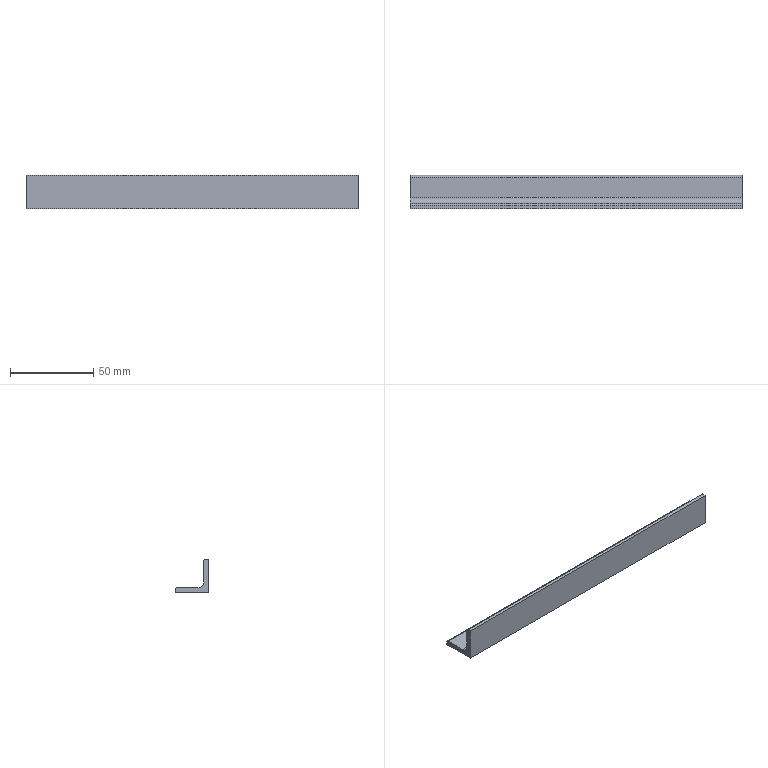Component | SolidWorks | hot-rolled equal angle gb-6 | 1 solid | 11 faces | box 200 x 20 x 20 mm | volume 22640 mm3 | plane 8 | cylinder 3 | commonest cylinder face diameters 2 x2 7 x1
build123d program:
from build123d import *

# Parameters (mm, degrees)
BASE_DEPTH = 200


with BuildPart() as part:
    # Sketch1 → Base (new body)
    with BuildSketch(Plane.YZ):
        with BuildLine():
            Line((0, 20), (0, 0))
            Line((0, 0), (20, 0))
            Line((20, 0), (20, 2))
            ThreePointArc((20, 2), (19.707, 2.707), (19, 3))
            Line((19, 3), (6.5, 3))
            ThreePointArc((6.5, 3), (4.025, 4.025), (3, 6.5))
            Line((3, 6.5), (3, 19))
            ThreePointArc((3, 19), (2.707, 19.707), (2, 20))
            Line((2, 20), (0, 20))
        make_face()
    extrude(amount=BASE_DEPTH)


solid = part.part

# Placed as in the assembly
solid = solid.moved(Location((-40, 537, -215), (0, 0, 0)))
STEP:
#1=CARTESIAN_POINT('',(-1.575,21.22,-7.677));
#2=VERTEX_POINT('',#1);
#3=CARTESIAN_POINT('',(-1.575,21.142,-7.677));
#4=VERTEX_POINT('',#3);
#5=CARTESIAN_POINT('',(-1.575,21.142,-7.677));
#6=DIRECTION('',(0.,-1.,-0.));
#7=VECTOR('',#6,39.37);
#8=LINE('',#5,#7);
#9=EDGE_CURVE('',#2,#4,#8,.T.);
#10=ORIENTED_EDGE('',*,*,#9,.T.);
#11=CARTESIAN_POINT('',(6.299,21.142,-7.677));
#12=VERTEX_POINT('',#11);
#13=CARTESIAN_POINT('',(6.299,21.142,-7.677));
#14=DIRECTION('',(-1.,0.,0.));
#15=VECTOR('',#14,39.37);
#16=LINE('',#13,#15);
#17=EDGE_CURVE('',#12,#4,#16,.T.);
#18=ORIENTED_EDGE('',*,*,#17,.F.);
#19=CARTESIAN_POINT('',(6.299,21.22,-7.677));
#20=VERTEX_POINT('',#19);
#21=CARTESIAN_POINT('',(6.299,21.142,-7.677));
#22=DIRECTION('',(0.,-1.,-0.));
#23=VECTOR('',#22,39.37);
#24=LINE('',#21,#23);
#25=EDGE_CURVE('',#20,#12,#24,.T.);
#26=ORIENTED_EDGE('',*,*,#25,.F.);
#27=CARTESIAN_POINT('',(6.299,21.22,-7.677));
#28=DIRECTION('',(-1.,0.,0.));
#29=VECTOR('',#28,39.37);
#30=LINE('',#27,#29);
#31=EDGE_CURVE('',#20,#2,#30,.T.);
#32=ORIENTED_EDGE('',*,*,#31,.T.);
#33=EDGE_LOOP('',(#10,#18,#26,#32));
#34=FACE_OUTER_BOUND('',#33,.T.);
#35=CARTESIAN_POINT('',(6.299,21.142,-7.677));
#36=DIRECTION('',(0.,0.,-1.));
#37=DIRECTION('',(0.,1.,0.));
#38=AXIS2_PLACEMENT_3D('',#35,#36,#37);
#39=PLANE('',#38);
#40=ADVANCED_FACE('',(#34),#39,.F.);
#41=CARTESIAN_POINT('',(-1.575,21.142,-8.465));
#42=VERTEX_POINT('',#41);
#43=CARTESIAN_POINT('',(-1.575,21.142,-7.677));
#44=DIRECTION('',(0.,-0.,-1.));
#45=VECTOR('',#44,39.37);
#46=LINE('',#43,#45);
#47=EDGE_CURVE('',#4,#42,#46,.T.);
#48=ORIENTED_EDGE('',*,*,#47,.T.);
#49=CARTESIAN_POINT('',(6.299,21.142,-8.465));
#50=VERTEX_POINT('',#49);
#51=CARTESIAN_POINT('',(6.299,21.142,-8.465));
#52=DIRECTION('',(-1.,0.,0.));
#53=VECTOR('',#52,39.37);
#54=LINE('',#51,#53);
#55=EDGE_CURVE('',#50,#42,#54,.T.);
#56=ORIENTED_EDGE('',*,*,#55,.F.);
#57=CARTESIAN_POINT('',(6.299,21.142,-7.677));
#58=DIRECTION('',(0.,-0.,-1.));
#59=VECTOR('',#58,39.37);
#60=LINE('',#57,#59);
#61=EDGE_CURVE('',#12,#50,#60,.T.);
#62=ORIENTED_EDGE('',*,*,#61,.F.);
#63=ORIENTED_EDGE('',*,*,#17,.T.);
#64=EDGE_LOOP('',(#48,#56,#62,#63));
#65=FACE_OUTER_BOUND('',#64,.T.);
#66=CARTESIAN_POINT('',(6.299,21.142,-7.677));
#67=DIRECTION('',(0.,1.,-0.));
#68=DIRECTION('',(0.,0.,1.));
#69=AXIS2_PLACEMENT_3D('',#66,#67,#68);
#70=PLANE('',#69);
#71=ADVANCED_FACE('',(#65),#70,.F.);
#72=CARTESIAN_POINT('',(-1.575,21.929,-8.465));
#73=VERTEX_POINT('',#72);
#74=CARTESIAN_POINT('',(-1.575,21.142,-8.465));
#75=DIRECTION('',(0.,1.,0.));
#76=VECTOR('',#75,39.37);
#77=LINE('',#74,#76);
#78=EDGE_CURVE('',#42,#73,#77,.T.);
#79=ORIENTED_EDGE('',*,*,#78,.T.);
#80=CARTESIAN_POINT('',(6.299,21.929,-8.465));
#81=VERTEX_POINT('',#80);
#82=CARTESIAN_POINT('',(6.299,21.929,-8.465));
#83=DIRECTION('',(-1.,0.,0.));
#84=VECTOR('',#83,39.37);
#85=LINE('',#82,#84);
#86=EDGE_CURVE('',#81,#73,#85,.T.);
#87=ORIENTED_EDGE('',*,*,#86,.F.);
#88=CARTESIAN_POINT('',(6.299,21.142,-8.465));
#89=DIRECTION('',(0.,1.,0.));
#90=VECTOR('',#89,39.37);
#91=LINE('',#88,#90);
#92=EDGE_CURVE('',#50,#81,#91,.T.);
#93=ORIENTED_EDGE('',*,*,#92,.F.);
#94=ORIENTED_EDGE('',*,*,#55,.T.);
#95=EDGE_LOOP('',(#79,#87,#93,#94));
#96=FACE_OUTER_BOUND('',#95,.T.);
#97=CARTESIAN_POINT('',(6.299,21.142,-8.465));
#98=DIRECTION('',(0.,0.,1.));
#99=DIRECTION('',(1.,0.,0.));
#100=AXIS2_PLACEMENT_3D('',#97,#98,#99);
#101=PLANE('',#100);
#102=ADVANCED_FACE('',(#96),#101,.F.);
#103=CARTESIAN_POINT('',(-1.575,21.929,-8.386));
#104=VERTEX_POINT('',#103);
#105=CARTESIAN_POINT('',(-1.575,21.929,-8.465));
#106=DIRECTION('',(0.,0.,1.));
#107=VECTOR('',#106,39.37);
#108=LINE('',#105,#107);
#109=EDGE_CURVE('',#73,#104,#108,.T.);
#110=ORIENTED_EDGE('',*,*,#109,.T.);
#111=CARTESIAN_POINT('',(6.299,21.929,-8.386));
#112=VERTEX_POINT('',#111);
#113=CARTESIAN_POINT('',(6.299,21.929,-8.386));
#114=DIRECTION('',(-1.,0.,0.));
#115=VECTOR('',#114,39.37);
#116=LINE('',#113,#115);
#117=EDGE_CURVE('',#112,#104,#116,.T.);
#118=ORIENTED_EDGE('',*,*,#117,.F.);
#119=CARTESIAN_POINT('',(6.299,21.929,-8.465));
#120=DIRECTION('',(0.,0.,1.));
#121=VECTOR('',#120,39.37);
#122=LINE('',#119,#121);
#123=EDGE_CURVE('',#81,#112,#122,.T.);
#124=ORIENTED_EDGE('',*,*,#123,.F.);
#125=ORIENTED_EDGE('',*,*,#86,.T.);
#126=EDGE_LOOP('',(#110,#118,#124,#125));
#127=FACE_OUTER_BOUND('',#126,.T.);
#128=CARTESIAN_POINT('',(6.299,21.929,-8.465));
#129=DIRECTION('',(0.,-1.,0.));
#130=DIRECTION('',(0.,-0.,-1.));
#131=AXIS2_PLACEMENT_3D('',#128,#129,#130);
#132=PLANE('',#131);
#133=ADVANCED_FACE('',(#127),#132,.F.);
#134=CARTESIAN_POINT('',(-1.575,21.89,-8.346));
#135=VERTEX_POINT('',#134);
#136=CARTESIAN_POINT('',(-1.575,21.89,-8.386));
#137=DIRECTION('',(1.,0.,0.));
#138=DIRECTION('',(0.,0.,-1.));
#139=AXIS2_PLACEMENT_3D('',#136,#137,#138);
#140=CIRCLE('',#139,0.03937);
#141=EDGE_CURVE('',#104,#135,#140,.T.);
#142=ORIENTED_EDGE('',*,*,#141,.T.);
#143=CARTESIAN_POINT('',(6.299,21.89,-8.346));
#144=VERTEX_POINT('',#143);
#145=CARTESIAN_POINT('',(6.299,21.89,-8.346));
#146=DIRECTION('',(-1.,0.,0.));
#147=VECTOR('',#146,39.37);
#148=LINE('',#145,#147);
#149=EDGE_CURVE('',#144,#135,#148,.T.);
#150=ORIENTED_EDGE('',*,*,#149,.F.);
#151=CARTESIAN_POINT('',(6.299,21.89,-8.386));
#152=DIRECTION('',(1.,0.,0.));
#153=DIRECTION('',(0.,0.,-1.));
#154=AXIS2_PLACEMENT_3D('',#151,#152,#153);
#155=CIRCLE('',#154,0.03937);
#156=EDGE_CURVE('',#112,#144,#155,.T.);
#157=ORIENTED_EDGE('',*,*,#156,.F.);
#158=ORIENTED_EDGE('',*,*,#117,.T.);
#159=EDGE_LOOP('',(#142,#150,#157,#158));
#160=FACE_OUTER_BOUND('',#159,.T.);
#161=CARTESIAN_POINT('',(6.299,21.89,-8.386));
#162=DIRECTION('',(-1.,0.,0.));
#163=DIRECTION('',(0.,0.,1.));
#164=AXIS2_PLACEMENT_3D('',#161,#162,#163);
#165=CYLINDRICAL_SURFACE('',#164,0.03937);
#166=ADVANCED_FACE('',(#160),#165,.T.);
#167=CARTESIAN_POINT('',(-1.575,21.398,-8.346));
#168=VERTEX_POINT('',#167);
#169=CARTESIAN_POINT('',(-1.575,21.398,-8.346));
#170=DIRECTION('',(0.,-1.,0.));
#171=VECTOR('',#170,39.37);
#172=LINE('',#169,#171);
#173=EDGE_CURVE('',#135,#168,#172,.T.);
#174=ORIENTED_EDGE('',*,*,#173,.T.);
#175=CARTESIAN_POINT('',(6.299,21.398,-8.346));
#176=VERTEX_POINT('',#175);
#177=CARTESIAN_POINT('',(6.299,21.398,-8.346));
#178=DIRECTION('',(-1.,0.,0.));
#179=VECTOR('',#178,39.37);
#180=LINE('',#177,#179);
#181=EDGE_CURVE('',#176,#168,#180,.T.);
#182=ORIENTED_EDGE('',*,*,#181,.F.);
#183=CARTESIAN_POINT('',(6.299,21.398,-8.346));
#184=DIRECTION('',(0.,-1.,0.));
#185=VECTOR('',#184,39.37);
#186=LINE('',#183,#185);
#187=EDGE_CURVE('',#144,#176,#186,.T.);
#188=ORIENTED_EDGE('',*,*,#187,.F.);
#189=ORIENTED_EDGE('',*,*,#149,.T.);
#190=EDGE_LOOP('',(#174,#182,#188,#189));
#191=FACE_OUTER_BOUND('',#190,.T.);
#192=CARTESIAN_POINT('',(6.299,21.398,-8.346));
#193=DIRECTION('',(0.,-0.,-1.));
#194=DIRECTION('',(0.,1.,-0.));
#195=AXIS2_PLACEMENT_3D('',#192,#193,#194);
#196=PLANE('',#195);
#197=ADVANCED_FACE('',(#191),#196,.F.);
#198=CARTESIAN_POINT('',(-1.575,21.26,-8.209));
#199=VERTEX_POINT('',#198);
#200=CARTESIAN_POINT('',(-1.575,21.398,-8.209));
#201=DIRECTION('',(-1.,0.,0.));
#202=DIRECTION('',(0.,0.,-1.));
#203=AXIS2_PLACEMENT_3D('',#200,#201,#202);
#204=CIRCLE('',#203,0.1378);
#205=EDGE_CURVE('',#168,#199,#204,.T.);
#206=ORIENTED_EDGE('',*,*,#205,.T.);
#207=CARTESIAN_POINT('',(6.299,21.26,-8.209));
#208=VERTEX_POINT('',#207);
#209=CARTESIAN_POINT('',(6.299,21.26,-8.209));
#210=DIRECTION('',(-1.,0.,0.));
#211=VECTOR('',#210,39.37);
#212=LINE('',#209,#211);
#213=EDGE_CURVE('',#208,#199,#212,.T.);
#214=ORIENTED_EDGE('',*,*,#213,.F.);
#215=CARTESIAN_POINT('',(6.299,21.398,-8.209));
#216=DIRECTION('',(-1.,0.,0.));
#217=DIRECTION('',(0.,0.,-1.));
#218=AXIS2_PLACEMENT_3D('',#215,#216,#217);
#219=CIRCLE('',#218,0.1378);
#220=EDGE_CURVE('',#176,#208,#219,.T.);
#221=ORIENTED_EDGE('',*,*,#220,.F.);
#222=ORIENTED_EDGE('',*,*,#181,.T.);
#223=EDGE_LOOP('',(#206,#214,#221,#222));
#224=FACE_OUTER_BOUND('',#223,.T.);
#225=CARTESIAN_POINT('',(6.299,21.398,-8.209));
#226=DIRECTION('',(-1.,0.,0.));
#227=DIRECTION('',(0.,0.,1.));
#228=AXIS2_PLACEMENT_3D('',#225,#226,#227);
#229=CYLINDRICAL_SURFACE('',#228,0.1378);
#230=ADVANCED_FACE('',(#224),#229,.F.);
#231=CARTESIAN_POINT('',(-1.575,21.26,-7.717));
#232=VERTEX_POINT('',#231);
#233=CARTESIAN_POINT('',(-1.575,21.26,-7.717));
#234=DIRECTION('',(0.,-0.,1.));
#235=VECTOR('',#234,39.37);
#236=LINE('',#233,#235);
#237=EDGE_CURVE('',#199,#232,#236,.T.);
#238=ORIENTED_EDGE('',*,*,#237,.T.);
#239=CARTESIAN_POINT('',(6.299,21.26,-7.717));
#240=VERTEX_POINT('',#239);
#241=CARTESIAN_POINT('',(6.299,21.26,-7.717));
#242=DIRECTION('',(-1.,0.,0.));
#243=VECTOR('',#242,39.37);
#244=LINE('',#241,#243);
#245=EDGE_CURVE('',#240,#232,#244,.T.);
#246=ORIENTED_EDGE('',*,*,#245,.F.);
#247=CARTESIAN_POINT('',(6.299,21.26,-7.717));
#248=DIRECTION('',(0.,-0.,1.));
#249=VECTOR('',#248,39.37);
#250=LINE('',#247,#249);
#251=EDGE_CURVE('',#208,#240,#250,.T.);
#252=ORIENTED_EDGE('',*,*,#251,.F.);
#253=ORIENTED_EDGE('',*,*,#213,.T.);
#254=EDGE_LOOP('',(#238,#246,#252,#253));
#255=FACE_OUTER_BOUND('',#254,.T.);
#256=CARTESIAN_POINT('',(6.299,21.26,-7.717));
#257=DIRECTION('',(0.,-1.,-0.));
#258=DIRECTION('',(0.,0.,-1.));
#259=AXIS2_PLACEMENT_3D('',#256,#257,#258);
#260=PLANE('',#259);
#261=ADVANCED_FACE('',(#255),#260,.F.);
#262=CARTESIAN_POINT('',(-1.575,21.22,-7.717));
#263=DIRECTION('',(1.,0.,0.));
#264=DIRECTION('',(0.,0.,1.));
#265=AXIS2_PLACEMENT_3D('',#262,#263,#264);
#266=CIRCLE('',#265,0.03937);
#267=EDGE_CURVE('',#232,#2,#266,.T.);
#268=ORIENTED_EDGE('',*,*,#267,.T.);
#269=ORIENTED_EDGE('',*,*,#31,.F.);
#270=CARTESIAN_POINT('',(6.299,21.22,-7.717));
#271=DIRECTION('',(1.,0.,0.));
#272=DIRECTION('',(0.,0.,1.));
#273=AXIS2_PLACEMENT_3D('',#270,#271,#272);
#274=CIRCLE('',#273,0.03937);
#275=EDGE_CURVE('',#240,#20,#274,.T.);
#276=ORIENTED_EDGE('',*,*,#275,.F.);
#277=ORIENTED_EDGE('',*,*,#245,.T.);
#278=EDGE_LOOP('',(#268,#269,#276,#277));
#279=FACE_OUTER_BOUND('',#278,.T.);
#280=CARTESIAN_POINT('',(6.299,21.22,-7.717));
#281=DIRECTION('',(-1.,0.,0.));
#282=DIRECTION('',(0.,0.,1.));
#283=AXIS2_PLACEMENT_3D('',#280,#281,#282);
#284=CYLINDRICAL_SURFACE('',#283,0.03937);
#285=ADVANCED_FACE('',(#279),#284,.T.);
#286=ORIENTED_EDGE('',*,*,#25,.T.);
#287=ORIENTED_EDGE('',*,*,#61,.T.);
#288=ORIENTED_EDGE('',*,*,#92,.T.);
#289=ORIENTED_EDGE('',*,*,#123,.T.);
#290=ORIENTED_EDGE('',*,*,#156,.T.);
#291=ORIENTED_EDGE('',*,*,#187,.T.);
#292=ORIENTED_EDGE('',*,*,#220,.T.);
#293=ORIENTED_EDGE('',*,*,#251,.T.);
#294=ORIENTED_EDGE('',*,*,#275,.T.);
#295=EDGE_LOOP('',(#286,#287,#288,#289,#290,#291,#292,#293,#294));
#296=FACE_OUTER_BOUND('',#295,.T.);
#297=CARTESIAN_POINT('',(6.299,21.22,-7.717));
#298=DIRECTION('',(-1.,0.,0.));
#299=DIRECTION('',(0.,0.,1.));
#300=AXIS2_PLACEMENT_3D('',#297,#298,#299);
#301=PLANE('',#300);
#302=ADVANCED_FACE('',(#296),#301,.F.);
#303=ORIENTED_EDGE('',*,*,#9,.F.);
#304=ORIENTED_EDGE('',*,*,#267,.F.);
#305=ORIENTED_EDGE('',*,*,#237,.F.);
#306=ORIENTED_EDGE('',*,*,#205,.F.);
#307=ORIENTED_EDGE('',*,*,#173,.F.);
#308=ORIENTED_EDGE('',*,*,#141,.F.);
#309=ORIENTED_EDGE('',*,*,#109,.F.);
#310=ORIENTED_EDGE('',*,*,#78,.F.);
#311=ORIENTED_EDGE('',*,*,#47,.F.);
#312=EDGE_LOOP('',(#303,#304,#305,#306,#307,#308,#309,#310,#311));
#313=FACE_OUTER_BOUND('',#312,.T.);
#314=CARTESIAN_POINT('',(-1.575,21.22,-7.717));
#315=DIRECTION('',(-1.,0.,0.));
#316=DIRECTION('',(0.,0.,1.));
#317=AXIS2_PLACEMENT_3D('',#314,#315,#316);
#318=PLANE('',#317);
#319=ADVANCED_FACE('',(#313),#318,.T.);
#320=CLOSED_SHELL('',(#40,#71,#102,#133,#166,#197,#230,#261,#285,#302,#319));
#321=MANIFOLD_SOLID_BREP('',#320);
#322=CARTESIAN_POINT('',(0.,0.,0.));
#323=DIRECTION('',(0.,0.,1.));
#324=DIRECTION('',(1.,0.,0.));
#325=AXIS2_PLACEMENT_3D('',#322,#323,#324);
#326=(LENGTH_UNIT()NAMED_UNIT(*)SI_UNIT($,.METRE.));
#327=LENGTH_MEASURE_WITH_UNIT(LENGTH_MEASURE(0.0254),#326);
#328=DIMENSIONAL_EXPONENTS(1.,0.,0.,0.,0.,0.,0.);
#329=(CONVERSION_BASED_UNIT('',#327)LENGTH_UNIT()NAMED_UNIT(#328));
#330=UNCERTAINTY_MEASURE_WITH_UNIT(LENGTH_MEASURE(0.00001),#329,'','');
#331=(NAMED_UNIT(*)PLANE_ANGLE_UNIT()SI_UNIT($,.RADIAN.));
#332=(NAMED_UNIT(*)SI_UNIT($,.STERADIAN.)SOLID_ANGLE_UNIT());
#333=(GEOMETRIC_REPRESENTATION_CONTEXT(3)GLOBAL_UNCERTAINTY_ASSIGNED_CONTEXT((#330))GLOBAL_UNIT_ASSIGNED_CONTEXT((#329,#331,#332))REPRESENTATION_CONTEXT('',''));
#334=ADVANCED_BREP_SHAPE_REPRESENTATION('',(#321,#325),#333);
#335=COLOUR_RGB('',0.7922,0.8196,0.9333);
#336=FILL_AREA_STYLE_COLOUR('',#335);
#337=FILL_AREA_STYLE('',(#336));
#338=SURFACE_STYLE_FILL_AREA(#337);
#339=SURFACE_SIDE_STYLE('',(#338));
#340=SURFACE_STYLE_USAGE(.BOTH.,#339);
#341=PRESENTATION_STYLE_ASSIGNMENT((#340));
#342=STYLED_ITEM('',(#341),#321);
#343=(LENGTH_UNIT()NAMED_UNIT(*)SI_UNIT($,.METRE.));
#344=LENGTH_MEASURE_WITH_UNIT(LENGTH_MEASURE(0.0254),#343);
#345=DIMENSIONAL_EXPONENTS(1.,0.,0.,0.,0.,0.,0.);
#346=(CONVERSION_BASED_UNIT('',#344)LENGTH_UNIT()NAMED_UNIT(#345));
#347=UNCERTAINTY_MEASURE_WITH_UNIT(LENGTH_MEASURE(0.00001),#346,'','');
#348=(NAMED_UNIT(*)PLANE_ANGLE_UNIT()SI_UNIT($,.RADIAN.));
#349=(NAMED_UNIT(*)SI_UNIT($,.STERADIAN.)SOLID_ANGLE_UNIT());
#350=(GEOMETRIC_REPRESENTATION_CONTEXT(3)GLOBAL_UNCERTAINTY_ASSIGNED_CONTEXT((#347))GLOBAL_UNIT_ASSIGNED_CONTEXT((#346,#348,#349))REPRESENTATION_CONTEXT('',''));
#351=MECHANICAL_DESIGN_GEOMETRIC_PRESENTATION_REPRESENTATION('',(#342),#350);
#352=PRESENTATION_LAYER_ASSIGNMENT('','',(#342));